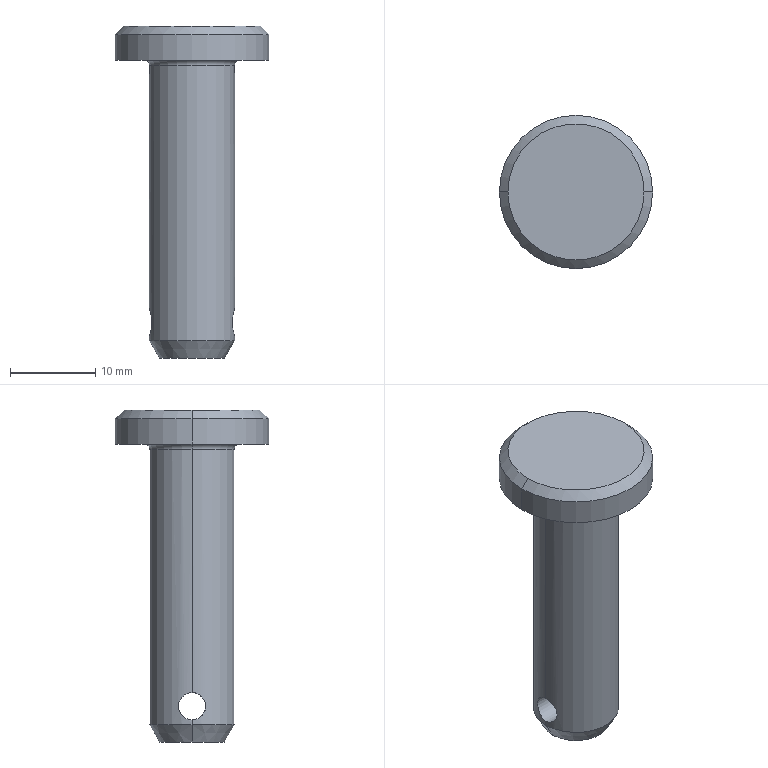Component | NX | GB_T_882_2008_PIN_A_TYPE_10X35 | 1 solid | 14 faces | volume 3629 mm3 | cylinder 5 | cone 4 | plane 3 | torus 2 | commonest cylinder face diameters 10 x2 18 x2 3.2 x1